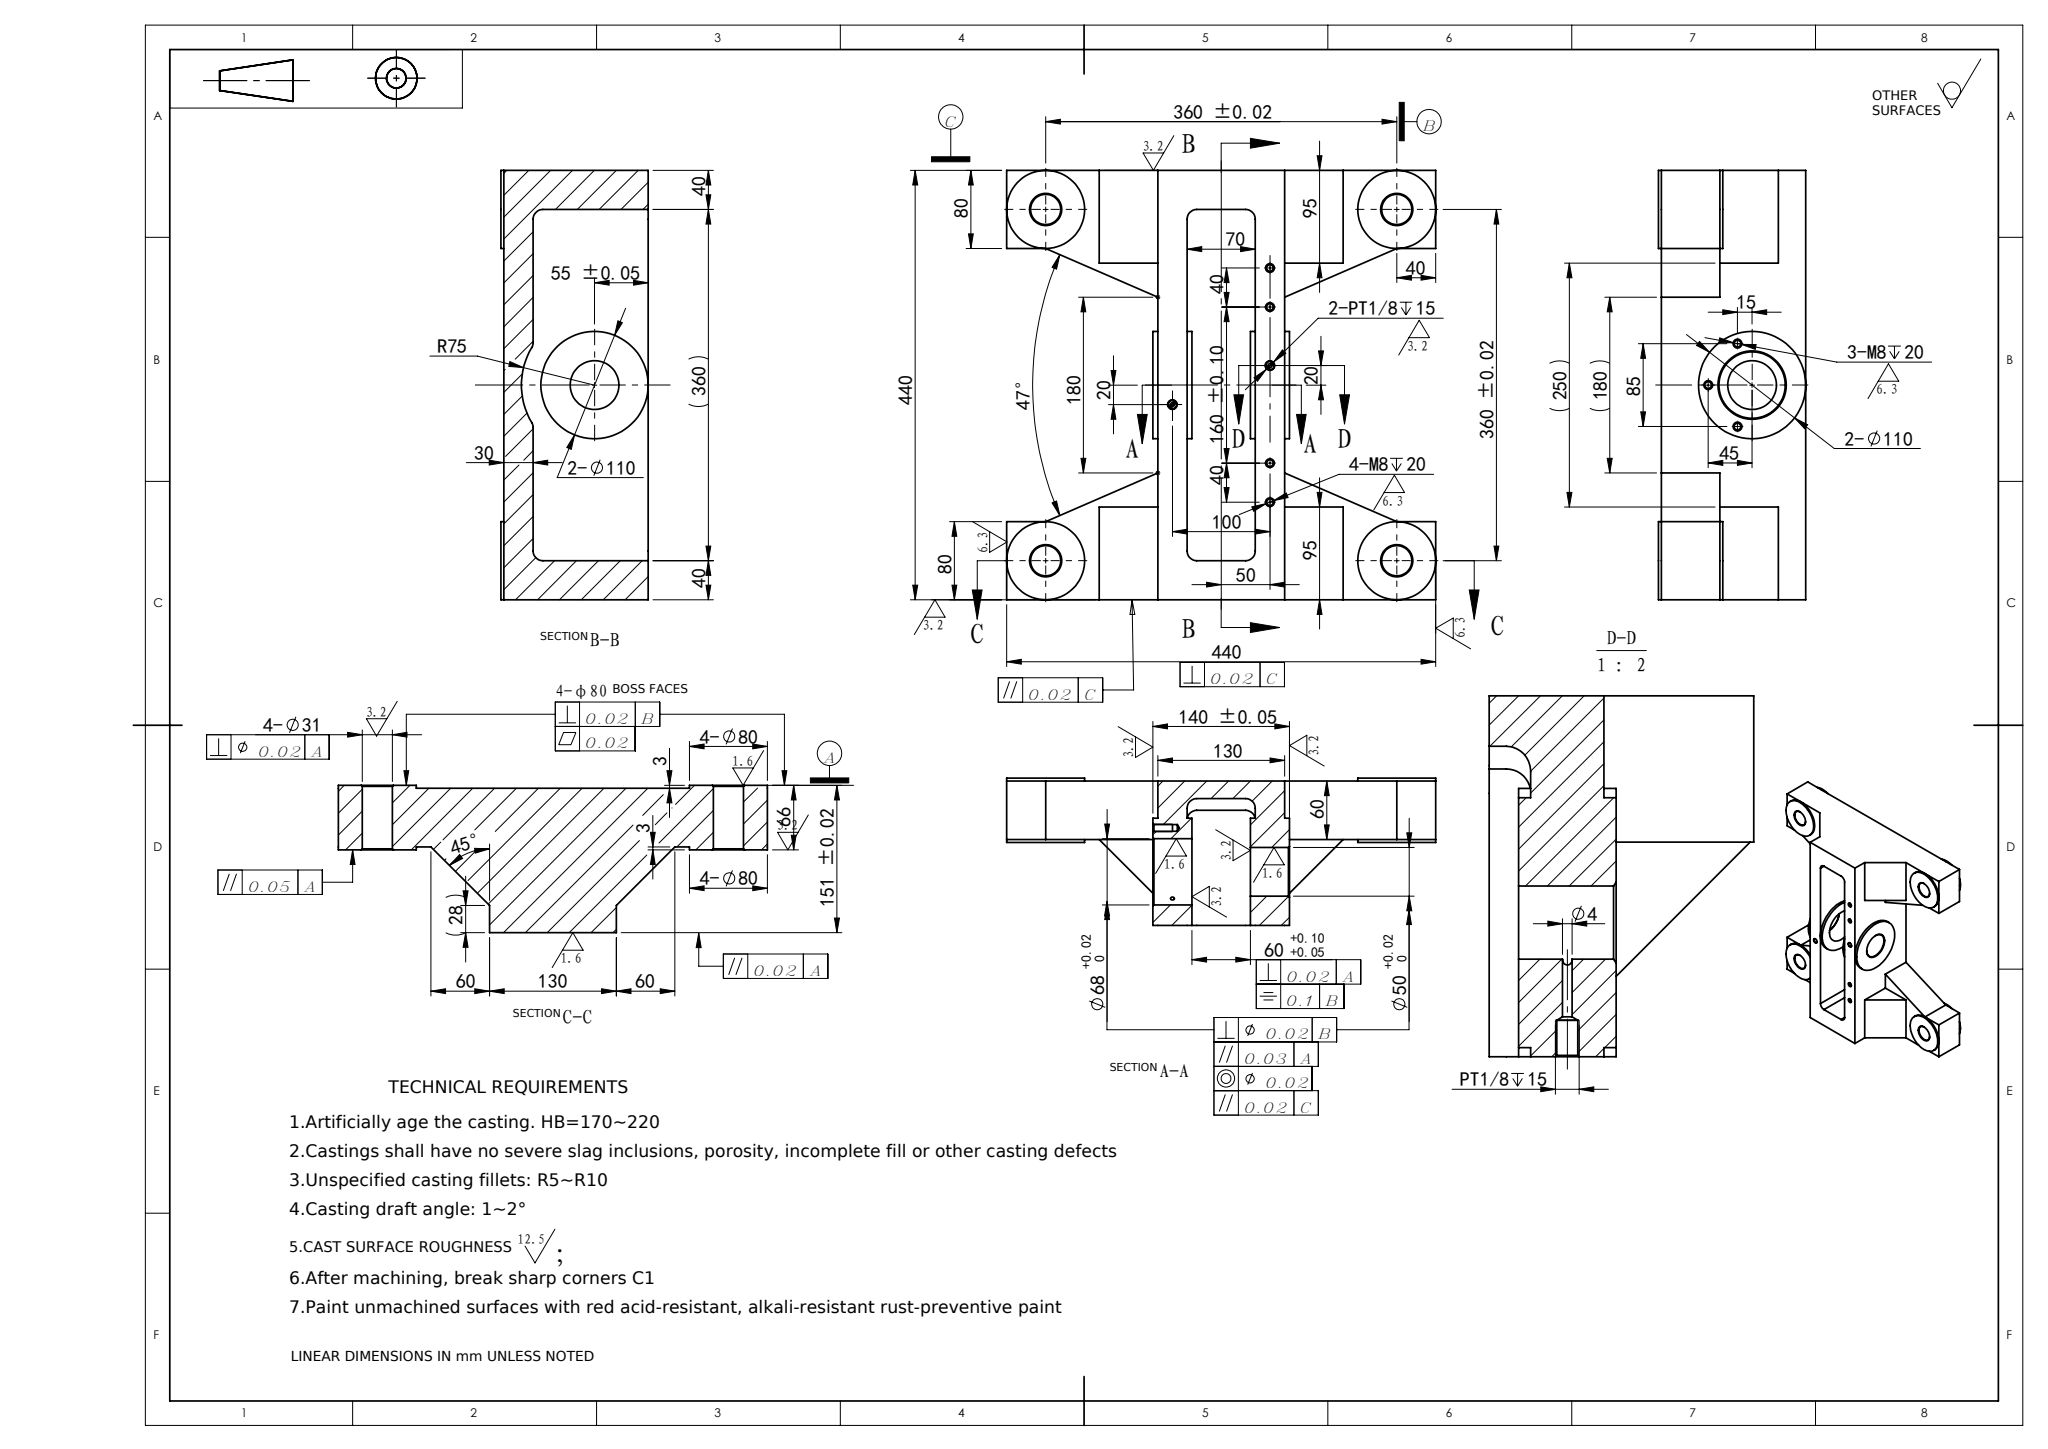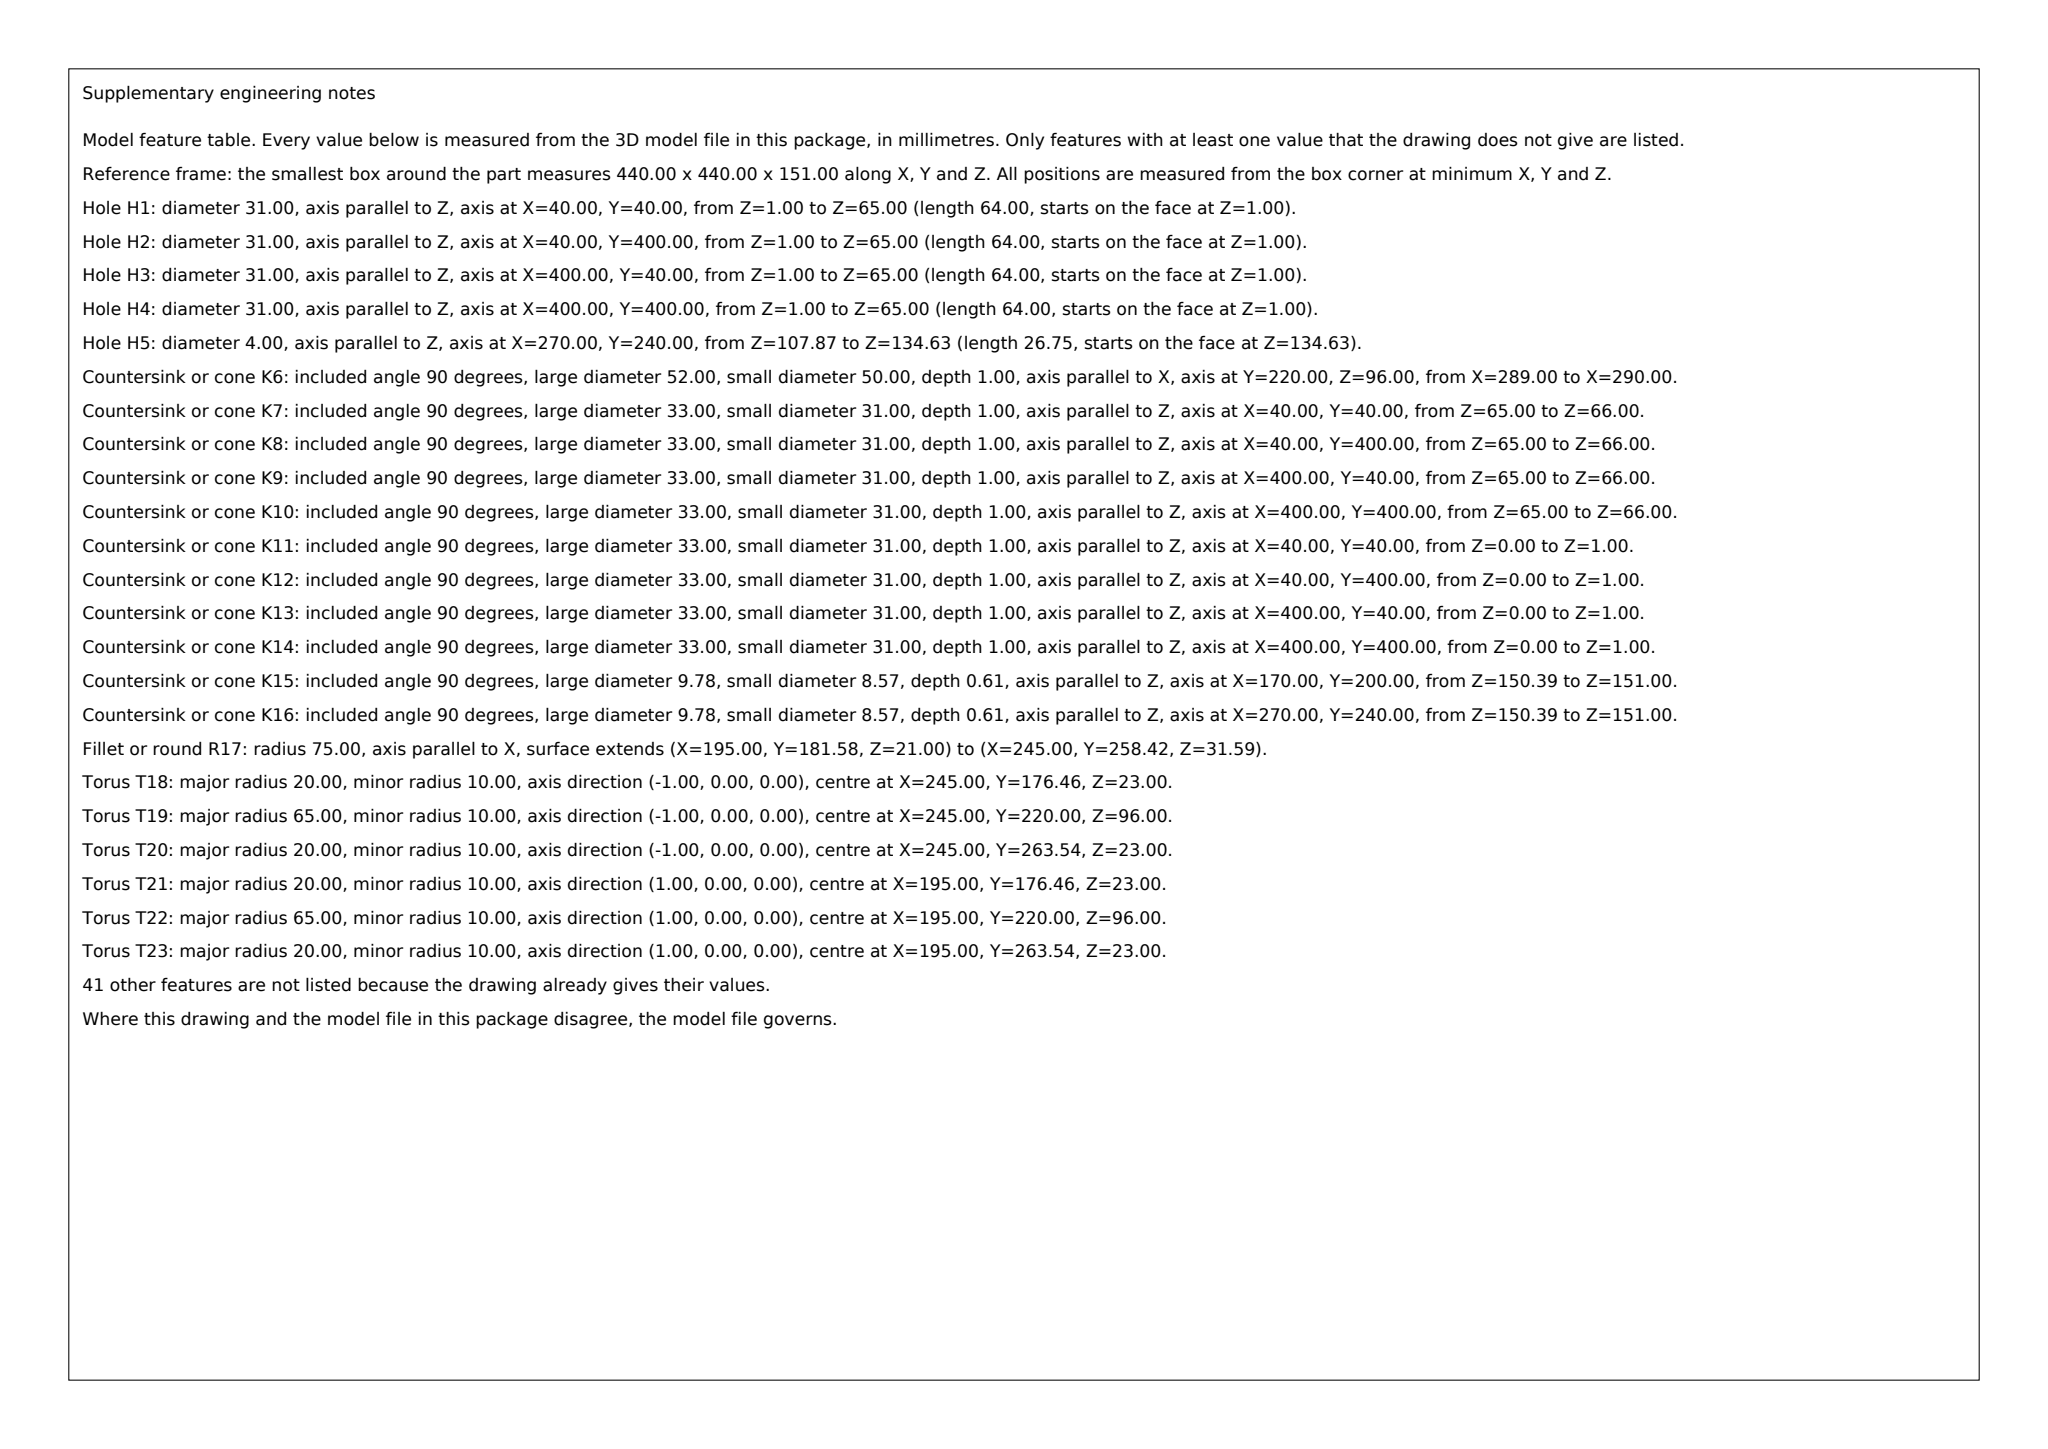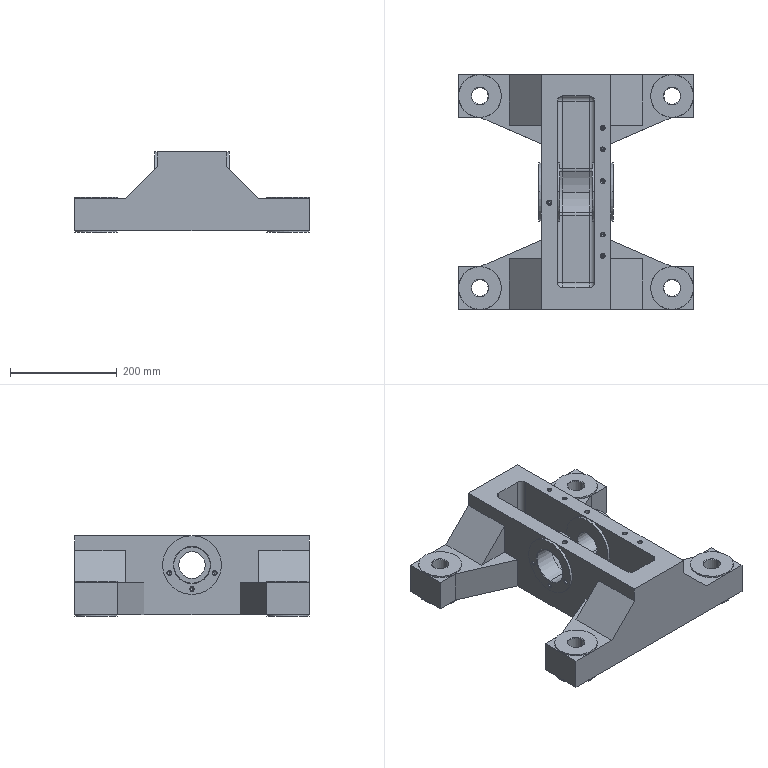Part | SolidWorks | mm | 1 solid | 202 faces | box 440 x 440 x 151 mm | volume 9702526 mm3 | cylinder 72 | plane 64 | cone 56 | torus 6 | sphere 4 | commonest cylinder face diameters 80 x16 6.8 x14 20 x12 110 x8 31 x8 8.566 x4 4 x4 50 x2